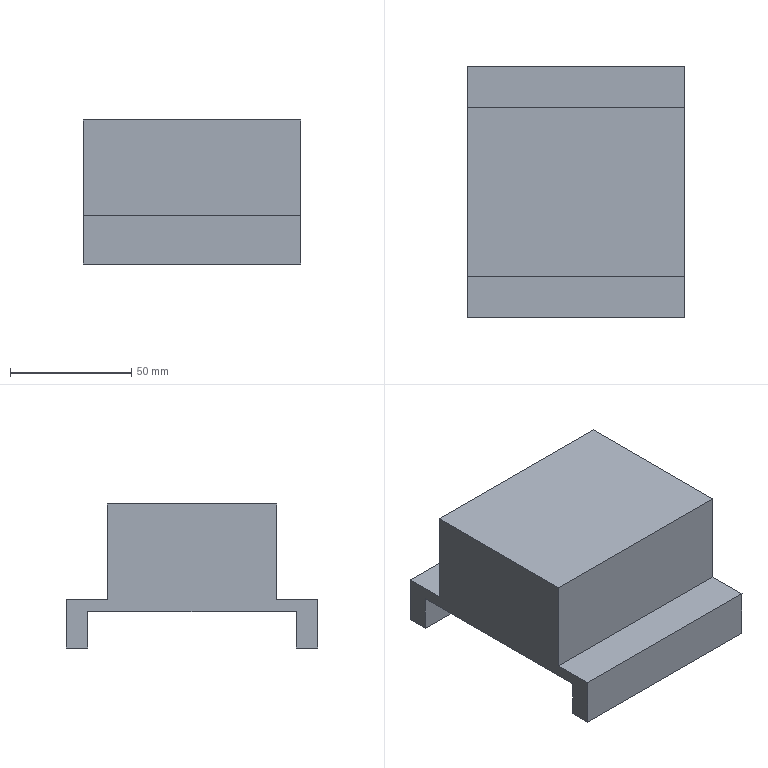Component | SolidWorks | X-AxisSlider-1 | 1 solid | 32 faces | box 90 x 104 x 59.5 mm | volume 318772 mm3 | plane 20 | cylinder 12 | commonest cylinder face diameters 5 x12
build123d program:
from build123d import *

# Parameters (mm, degrees)
BOSS_EXTRUDE1_DEPTH = 90
SKETCH3_R           = 2.5
CUT_EXTRUDE1_DEPTH  = 10


with BuildPart() as part:
    # Sketch2 → Boss-Extrude1 (new body)
    with BuildSketch(Plane.XY):
        Polygon((-35, 0), (35, 0), (35, 39.5), (52, 39.5), (52, 59.5), (43, 59.5), (43, 44.5), (-43, 44.5), (-43, 59.5), (-52, 59.5), (-52, 39.5), (-35, 39.5), align=None)
    extrude(amount=BOSS_EXTRUDE1_DEPTH)

    # Sketch3 → Cut-Extrude1 (cut)
    with BuildSketch(Plane(origin=(0, 59.5, 0), x_dir=(1, 0, 0), z_dir=(0, 1, 0))):
        with Locations(Location((-47.5, -8, 0), (0, 0, 180))):
            Circle(SKETCH3_R)
        with Locations(Location((-47.5, -45, 0), (0, 0, 180))):
            Circle(SKETCH3_R)
        with Locations(Location((-47.5, -82, 0), (0, 0, 180))):
            Circle(SKETCH3_R)
        with Locations(Location((47.5, -8, 0), (0, 0, 180))):
            Circle(SKETCH3_R)
        with Locations(Location((47.5, -45, 0), (0, 0, 180))):
            Circle(SKETCH3_R)
        with Locations(Location((47.5, -82, 0), (0, 0, 180))):
            Circle(SKETCH3_R)
    extrude(amount=-CUT_EXTRUDE1_DEPTH, mode=Mode.SUBTRACT)


solid = part.part

# Placed as in the assembly
solid = solid.moved(Location((-25.771, 0, 59), (-90, 90, 0)))
STEP:
#1=COLOUR_RGB('',0.7922,0.8196,0.9333);
#2=FILL_AREA_STYLE_COLOUR('',#1);
#3=FILL_AREA_STYLE('',(#2));
#4=SURFACE_STYLE_FILL_AREA(#3);
#5=SURFACE_SIDE_STYLE('',(#4));
#6=SURFACE_STYLE_USAGE(.BOTH.,#5);
#7=PRESENTATION_STYLE_ASSIGNMENT((#6));
#8=CARTESIAN_POINT('',(2.214,-1.969,0.374));
#9=VERTEX_POINT('',#8);
#10=CARTESIAN_POINT('',(2.214,-1.772,0.374));
#11=VERTEX_POINT('',#10);
#12=CARTESIAN_POINT('',(2.214,-1.87,0.374));
#13=DIRECTION('',(0.,0.,-1.));
#14=DIRECTION('',(0.,1.,0.));
#15=AXIS2_PLACEMENT_3D('',#12,#13,#14);
#16=CIRCLE('',#15,0.09843);
#17=EDGE_CURVE('',#9,#11,#16,.T.);
#18=ORIENTED_EDGE('',*,*,#17,.F.);
#19=CARTESIAN_POINT('',(2.214,-1.969,-0.01969));
#20=VERTEX_POINT('',#19);
#21=CARTESIAN_POINT('',(2.214,-1.969,0.374));
#22=DIRECTION('',(0.,0.,-1.));
#23=VECTOR('',#22,39.37);
#24=LINE('',#21,#23);
#25=EDGE_CURVE('',#9,#20,#24,.T.);
#26=ORIENTED_EDGE('',*,*,#25,.T.);
#27=CARTESIAN_POINT('',(2.214,-1.772,-0.01969));
#28=VERTEX_POINT('',#27);
#29=CARTESIAN_POINT('',(2.214,-1.87,-0.01969));
#30=DIRECTION('',(0.,0.,-1.));
#31=DIRECTION('',(0.,1.,0.));
#32=AXIS2_PLACEMENT_3D('',#29,#30,#31);
#33=CIRCLE('',#32,0.09843);
#34=EDGE_CURVE('',#20,#28,#33,.T.);
#35=ORIENTED_EDGE('',*,*,#34,.T.);
#36=CARTESIAN_POINT('',(2.214,-1.772,0.374));
#37=DIRECTION('',(0.,0.,-1.));
#38=VECTOR('',#37,39.37);
#39=LINE('',#36,#38);
#40=EDGE_CURVE('',#11,#28,#39,.T.);
#41=ORIENTED_EDGE('',*,*,#40,.F.);
#42=EDGE_LOOP('',(#18,#26,#35,#41));
#43=FACE_OUTER_BOUND('',#42,.T.);
#44=CARTESIAN_POINT('',(2.214,-1.87,0.374));
#45=DIRECTION('',(0.,0.,-1.));
#46=DIRECTION('',(0.,1.,0.));
#47=AXIS2_PLACEMENT_3D('',#44,#45,#46);
#48=CYLINDRICAL_SURFACE('',#47,0.09843);
#49=ADVANCED_FACE('',(#43),#48,.F.);
#50=CARTESIAN_POINT('',(0.7571,-1.969,0.374));
#51=VERTEX_POINT('',#50);
#52=CARTESIAN_POINT('',(0.7571,-1.772,0.374));
#53=VERTEX_POINT('',#52);
#54=CARTESIAN_POINT('',(0.7571,-1.87,0.374));
#55=DIRECTION('',(0.,0.,-1.));
#56=DIRECTION('',(0.,1.,0.));
#57=AXIS2_PLACEMENT_3D('',#54,#55,#56);
#58=CIRCLE('',#57,0.09843);
#59=EDGE_CURVE('',#51,#53,#58,.T.);
#60=ORIENTED_EDGE('',*,*,#59,.F.);
#61=CARTESIAN_POINT('',(0.7571,-1.969,-0.01969));
#62=VERTEX_POINT('',#61);
#63=CARTESIAN_POINT('',(0.7571,-1.969,0.374));
#64=DIRECTION('',(0.,0.,-1.));
#65=VECTOR('',#64,39.37);
#66=LINE('',#63,#65);
#67=EDGE_CURVE('',#51,#62,#66,.T.);
#68=ORIENTED_EDGE('',*,*,#67,.T.);
#69=CARTESIAN_POINT('',(0.7571,-1.772,-0.01969));
#70=VERTEX_POINT('',#69);
#71=CARTESIAN_POINT('',(0.7571,-1.87,-0.01969));
#72=DIRECTION('',(0.,0.,-1.));
#73=DIRECTION('',(0.,1.,0.));
#74=AXIS2_PLACEMENT_3D('',#71,#72,#73);
#75=CIRCLE('',#74,0.09843);
#76=EDGE_CURVE('',#62,#70,#75,.T.);
#77=ORIENTED_EDGE('',*,*,#76,.T.);
#78=CARTESIAN_POINT('',(0.7571,-1.772,0.374));
#79=DIRECTION('',(0.,0.,-1.));
#80=VECTOR('',#79,39.37);
#81=LINE('',#78,#80);
#82=EDGE_CURVE('',#53,#70,#81,.T.);
#83=ORIENTED_EDGE('',*,*,#82,.F.);
#84=EDGE_LOOP('',(#60,#68,#77,#83));
#85=FACE_OUTER_BOUND('',#84,.T.);
#86=CARTESIAN_POINT('',(0.7571,-1.87,0.374));
#87=DIRECTION('',(0.,0.,-1.));
#88=DIRECTION('',(0.,1.,0.));
#89=AXIS2_PLACEMENT_3D('',#86,#87,#88);
#90=CYLINDRICAL_SURFACE('',#89,0.09843);
#91=ADVANCED_FACE('',(#85),#90,.F.);
#92=CARTESIAN_POINT('',(-0.6996,-1.969,0.374));
#93=VERTEX_POINT('',#92);
#94=CARTESIAN_POINT('',(-0.6996,-1.772,0.374));
#95=VERTEX_POINT('',#94);
#96=CARTESIAN_POINT('',(-0.6996,-1.87,0.374));
#97=DIRECTION('',(0.,0.,-1.));
#98=DIRECTION('',(0.,1.,0.));
#99=AXIS2_PLACEMENT_3D('',#96,#97,#98);
#100=CIRCLE('',#99,0.09843);
#101=EDGE_CURVE('',#93,#95,#100,.T.);
#102=ORIENTED_EDGE('',*,*,#101,.F.);
#103=CARTESIAN_POINT('',(-0.6996,-1.969,-0.01969));
#104=VERTEX_POINT('',#103);
#105=CARTESIAN_POINT('',(-0.6996,-1.969,0.374));
#106=DIRECTION('',(0.,0.,-1.));
#107=VECTOR('',#106,39.37);
#108=LINE('',#105,#107);
#109=EDGE_CURVE('',#93,#104,#108,.T.);
#110=ORIENTED_EDGE('',*,*,#109,.T.);
#111=CARTESIAN_POINT('',(-0.6996,-1.772,-0.01969));
#112=VERTEX_POINT('',#111);
#113=CARTESIAN_POINT('',(-0.6996,-1.87,-0.01969));
#114=DIRECTION('',(0.,0.,-1.));
#115=DIRECTION('',(0.,1.,0.));
#116=AXIS2_PLACEMENT_3D('',#113,#114,#115);
#117=CIRCLE('',#116,0.09843);
#118=EDGE_CURVE('',#104,#112,#117,.T.);
#119=ORIENTED_EDGE('',*,*,#118,.T.);
#120=CARTESIAN_POINT('',(-0.6996,-1.772,0.374));
#121=DIRECTION('',(0.,0.,-1.));
#122=VECTOR('',#121,39.37);
#123=LINE('',#120,#122);
#124=EDGE_CURVE('',#95,#112,#123,.T.);
#125=ORIENTED_EDGE('',*,*,#124,.F.);
#126=EDGE_LOOP('',(#102,#110,#119,#125));
#127=FACE_OUTER_BOUND('',#126,.T.);
#128=CARTESIAN_POINT('',(-0.6996,-1.87,0.374));
#129=DIRECTION('',(0.,0.,-1.));
#130=DIRECTION('',(0.,1.,0.));
#131=AXIS2_PLACEMENT_3D('',#128,#129,#130);
#132=CYLINDRICAL_SURFACE('',#131,0.09843);
#133=ADVANCED_FACE('',(#127),#132,.F.);
#134=CARTESIAN_POINT('',(2.214,1.772,0.374));
#135=VERTEX_POINT('',#134);
#136=CARTESIAN_POINT('',(2.214,1.969,0.374));
#137=VERTEX_POINT('',#136);
#138=CARTESIAN_POINT('',(2.214,1.87,0.374));
#139=DIRECTION('',(0.,0.,-1.));
#140=DIRECTION('',(0.,1.,0.));
#141=AXIS2_PLACEMENT_3D('',#138,#139,#140);
#142=CIRCLE('',#141,0.09843);
#143=EDGE_CURVE('',#135,#137,#142,.T.);
#144=ORIENTED_EDGE('',*,*,#143,.F.);
#145=CARTESIAN_POINT('',(2.214,1.772,-0.01969));
#146=VERTEX_POINT('',#145);
#147=CARTESIAN_POINT('',(2.214,1.772,0.374));
#148=DIRECTION('',(0.,0.,-1.));
#149=VECTOR('',#148,39.37);
#150=LINE('',#147,#149);
#151=EDGE_CURVE('',#135,#146,#150,.T.);
#152=ORIENTED_EDGE('',*,*,#151,.T.);
#153=CARTESIAN_POINT('',(2.214,1.969,-0.01969));
#154=VERTEX_POINT('',#153);
#155=CARTESIAN_POINT('',(2.214,1.87,-0.01969));
#156=DIRECTION('',(0.,0.,-1.));
#157=DIRECTION('',(0.,1.,0.));
#158=AXIS2_PLACEMENT_3D('',#155,#156,#157);
#159=CIRCLE('',#158,0.09843);
#160=EDGE_CURVE('',#146,#154,#159,.T.);
#161=ORIENTED_EDGE('',*,*,#160,.T.);
#162=CARTESIAN_POINT('',(2.214,1.969,0.374));
#163=DIRECTION('',(0.,0.,-1.));
#164=VECTOR('',#163,39.37);
#165=LINE('',#162,#164);
#166=EDGE_CURVE('',#137,#154,#165,.T.);
#167=ORIENTED_EDGE('',*,*,#166,.F.);
#168=EDGE_LOOP('',(#144,#152,#161,#167));
#169=FACE_OUTER_BOUND('',#168,.T.);
#170=CARTESIAN_POINT('',(2.214,1.87,0.374));
#171=DIRECTION('',(0.,0.,-1.));
#172=DIRECTION('',(0.,1.,0.));
#173=AXIS2_PLACEMENT_3D('',#170,#171,#172);
#174=CYLINDRICAL_SURFACE('',#173,0.09843);
#175=ADVANCED_FACE('',(#169),#174,.F.);
#176=CARTESIAN_POINT('',(0.7571,1.772,0.374));
#177=VERTEX_POINT('',#176);
#178=CARTESIAN_POINT('',(0.7571,1.969,0.374));
#179=VERTEX_POINT('',#178);
#180=CARTESIAN_POINT('',(0.7571,1.87,0.374));
#181=DIRECTION('',(0.,0.,-1.));
#182=DIRECTION('',(0.,1.,0.));
#183=AXIS2_PLACEMENT_3D('',#180,#181,#182);
#184=CIRCLE('',#183,0.09843);
#185=EDGE_CURVE('',#177,#179,#184,.T.);
#186=ORIENTED_EDGE('',*,*,#185,.F.);
#187=CARTESIAN_POINT('',(0.7571,1.772,-0.01969));
#188=VERTEX_POINT('',#187);
#189=CARTESIAN_POINT('',(0.7571,1.772,0.374));
#190=DIRECTION('',(0.,0.,-1.));
#191=VECTOR('',#190,39.37);
#192=LINE('',#189,#191);
#193=EDGE_CURVE('',#177,#188,#192,.T.);
#194=ORIENTED_EDGE('',*,*,#193,.T.);
#195=CARTESIAN_POINT('',(0.7571,1.969,-0.01969));
#196=VERTEX_POINT('',#195);
#197=CARTESIAN_POINT('',(0.7571,1.87,-0.01969));
#198=DIRECTION('',(0.,0.,-1.));
#199=DIRECTION('',(0.,1.,0.));
#200=AXIS2_PLACEMENT_3D('',#197,#198,#199);
#201=CIRCLE('',#200,0.09843);
#202=EDGE_CURVE('',#188,#196,#201,.T.);
#203=ORIENTED_EDGE('',*,*,#202,.T.);
#204=CARTESIAN_POINT('',(0.7571,1.969,0.374));
#205=DIRECTION('',(0.,0.,-1.));
#206=VECTOR('',#205,39.37);
#207=LINE('',#204,#206);
#208=EDGE_CURVE('',#179,#196,#207,.T.);
#209=ORIENTED_EDGE('',*,*,#208,.F.);
#210=EDGE_LOOP('',(#186,#194,#203,#209));
#211=FACE_OUTER_BOUND('',#210,.T.);
#212=CARTESIAN_POINT('',(0.7571,1.87,0.374));
#213=DIRECTION('',(0.,0.,-1.));
#214=DIRECTION('',(0.,1.,0.));
#215=AXIS2_PLACEMENT_3D('',#212,#213,#214);
#216=CYLINDRICAL_SURFACE('',#215,0.09843);
#217=ADVANCED_FACE('',(#211),#216,.F.);
#218=CARTESIAN_POINT('',(-0.6996,1.772,0.374));
#219=VERTEX_POINT('',#218);
#220=CARTESIAN_POINT('',(-0.6996,1.969,0.374));
#221=VERTEX_POINT('',#220);
#222=CARTESIAN_POINT('',(-0.6996,1.87,0.374));
#223=DIRECTION('',(0.,0.,-1.));
#224=DIRECTION('',(0.,1.,0.));
#225=AXIS2_PLACEMENT_3D('',#222,#223,#224);
#226=CIRCLE('',#225,0.09843);
#227=EDGE_CURVE('',#219,#221,#226,.T.);
#228=ORIENTED_EDGE('',*,*,#227,.F.);
#229=CARTESIAN_POINT('',(-0.6996,1.772,-0.01969));
#230=VERTEX_POINT('',#229);
#231=CARTESIAN_POINT('',(-0.6996,1.772,0.374));
#232=DIRECTION('',(0.,0.,-1.));
#233=VECTOR('',#232,39.37);
#234=LINE('',#231,#233);
#235=EDGE_CURVE('',#219,#230,#234,.T.);
#236=ORIENTED_EDGE('',*,*,#235,.T.);
#237=CARTESIAN_POINT('',(-0.6996,1.969,-0.01969));
#238=VERTEX_POINT('',#237);
#239=CARTESIAN_POINT('',(-0.6996,1.87,-0.01969));
#240=DIRECTION('',(0.,0.,-1.));
#241=DIRECTION('',(0.,1.,0.));
#242=AXIS2_PLACEMENT_3D('',#239,#240,#241);
#243=CIRCLE('',#242,0.09843);
#244=EDGE_CURVE('',#230,#238,#243,.T.);
#245=ORIENTED_EDGE('',*,*,#244,.T.);
#246=CARTESIAN_POINT('',(-0.6996,1.969,0.374));
#247=DIRECTION('',(0.,0.,-1.));
#248=VECTOR('',#247,39.37);
#249=LINE('',#246,#248);
#250=EDGE_CURVE('',#221,#238,#249,.T.);
#251=ORIENTED_EDGE('',*,*,#250,.F.);
#252=EDGE_LOOP('',(#228,#236,#245,#251));
#253=FACE_OUTER_BOUND('',#252,.T.);
#254=CARTESIAN_POINT('',(-0.6996,1.87,0.374));
#255=DIRECTION('',(0.,0.,-1.));
#256=DIRECTION('',(0.,1.,0.));
#257=AXIS2_PLACEMENT_3D('',#254,#255,#256);
#258=CYLINDRICAL_SURFACE('',#257,0.09843);
#259=ADVANCED_FACE('',(#253),#258,.F.);
#260=CARTESIAN_POINT('',(-1.015,1.378,0.7677));
#261=VERTEX_POINT('',#260);
#262=CARTESIAN_POINT('',(-1.015,1.378,2.323));
#263=VERTEX_POINT('',#262);
#264=CARTESIAN_POINT('',(-1.015,1.378,2.323));
#265=DIRECTION('',(-0.,-0.,1.));
#266=VECTOR('',#265,39.37);
#267=LINE('',#264,#266);
#268=EDGE_CURVE('',#261,#263,#267,.T.);
#269=ORIENTED_EDGE('',*,*,#268,.T.);
#270=CARTESIAN_POINT('',(2.529,1.378,2.323));
#271=VERTEX_POINT('',#270);
#272=CARTESIAN_POINT('',(2.529,1.378,2.323));
#273=DIRECTION('',(-1.,-0.,-0.));
#274=VECTOR('',#273,39.37);
#275=LINE('',#272,#274);
#276=EDGE_CURVE('',#271,#263,#275,.T.);
#277=ORIENTED_EDGE('',*,*,#276,.F.);
#278=CARTESIAN_POINT('',(2.529,1.378,0.7677));
#279=VERTEX_POINT('',#278);
#280=CARTESIAN_POINT('',(2.529,1.378,2.323));
#281=DIRECTION('',(-0.,-0.,1.));
#282=VECTOR('',#281,39.37);
#283=LINE('',#280,#282);
#284=EDGE_CURVE('',#279,#271,#283,.T.);
#285=ORIENTED_EDGE('',*,*,#284,.F.);
#286=CARTESIAN_POINT('',(2.529,1.378,0.7677));
#287=DIRECTION('',(-1.,-0.,-0.));
#288=VECTOR('',#287,39.37);
#289=LINE('',#286,#288);
#290=EDGE_CURVE('',#279,#261,#289,.T.);
#291=ORIENTED_EDGE('',*,*,#290,.T.);
#292=EDGE_LOOP('',(#269,#277,#285,#291));
#293=FACE_OUTER_BOUND('',#292,.T.);
#294=CARTESIAN_POINT('',(2.529,1.378,2.323));
#295=DIRECTION('',(0.,-1.,-0.));
#296=DIRECTION('',(-1.,-0.,-0.));
#297=AXIS2_PLACEMENT_3D('',#294,#295,#296);
#298=PLANE('',#297);
#299=ADVANCED_FACE('',(#293),#298,.F.);
#300=CARTESIAN_POINT('',(-1.015,-1.378,2.323));
#301=VERTEX_POINT('',#300);
#302=CARTESIAN_POINT('',(-1.015,1.378,2.323));
#303=DIRECTION('',(0.,-1.,-0.));
#304=VECTOR('',#303,39.37);
#305=LINE('',#302,#304);
#306=EDGE_CURVE('',#263,#301,#305,.T.);
#307=ORIENTED_EDGE('',*,*,#306,.T.);
#308=CARTESIAN_POINT('',(2.529,-1.378,2.323));
#309=VERTEX_POINT('',#308);
#310=CARTESIAN_POINT('',(2.529,-1.378,2.323));
#311=DIRECTION('',(-1.,-0.,-0.));
#312=VECTOR('',#311,39.37);
#313=LINE('',#310,#312);
#314=EDGE_CURVE('',#309,#301,#313,.T.);
#315=ORIENTED_EDGE('',*,*,#314,.F.);
#316=CARTESIAN_POINT('',(2.529,1.378,2.323));
#317=DIRECTION('',(0.,-1.,-0.));
#318=VECTOR('',#317,39.37);
#319=LINE('',#316,#318);
#320=EDGE_CURVE('',#271,#309,#319,.T.);
#321=ORIENTED_EDGE('',*,*,#320,.F.);
#322=ORIENTED_EDGE('',*,*,#276,.T.);
#323=EDGE_LOOP('',(#307,#315,#321,#322));
#324=FACE_OUTER_BOUND('',#323,.T.);
#325=CARTESIAN_POINT('',(2.529,1.378,2.323));
#326=DIRECTION('',(0.,0.,-1.));
#327=DIRECTION('',(1.,0.,0.));
#328=AXIS2_PLACEMENT_3D('',#325,#326,#327);
#329=PLANE('',#328);
#330=ADVANCED_FACE('',(#324),#329,.F.);
#331=CARTESIAN_POINT('',(-1.015,-1.378,0.7677));
#332=VERTEX_POINT('',#331);
#333=CARTESIAN_POINT('',(-1.015,-1.378,2.323));
#334=DIRECTION('',(0.,0.,-1.));
#335=VECTOR('',#334,39.37);
#336=LINE('',#333,#335);
#337=EDGE_CURVE('',#301,#332,#336,.T.);
#338=ORIENTED_EDGE('',*,*,#337,.T.);
#339=CARTESIAN_POINT('',(2.529,-1.378,0.7677));
#340=VERTEX_POINT('',#339);
#341=CARTESIAN_POINT('',(2.529,-1.378,0.7677));
#342=DIRECTION('',(-1.,-0.,-0.));
#343=VECTOR('',#342,39.37);
#344=LINE('',#341,#343);
#345=EDGE_CURVE('',#340,#332,#344,.T.);
#346=ORIENTED_EDGE('',*,*,#345,.F.);
#347=CARTESIAN_POINT('',(2.529,-1.378,2.323));
#348=DIRECTION('',(0.,0.,-1.));
#349=VECTOR('',#348,39.37);
#350=LINE('',#347,#349);
#351=EDGE_CURVE('',#309,#340,#350,.T.);
#352=ORIENTED_EDGE('',*,*,#351,.F.);
#353=ORIENTED_EDGE('',*,*,#314,.T.);
#354=EDGE_LOOP('',(#338,#346,#352,#353));
#355=FACE_OUTER_BOUND('',#354,.T.);
#356=CARTESIAN_POINT('',(2.529,-1.378,2.323));
#357=DIRECTION('',(-0.,1.,0.));
#358=DIRECTION('',(1.,0.,0.));
#359=AXIS2_PLACEMENT_3D('',#356,#357,#358);
#360=PLANE('',#359);
#361=ADVANCED_FACE('',(#355),#360,.F.);
#362=CARTESIAN_POINT('',(-1.015,-2.047,0.7677));
#363=VERTEX_POINT('',#362);
#364=CARTESIAN_POINT('',(-1.015,-1.378,0.7677));
#365=DIRECTION('',(0.,-1.,-0.));
#366=VECTOR('',#365,39.37);
#367=LINE('',#364,#366);
#368=EDGE_CURVE('',#332,#363,#367,.T.);
#369=ORIENTED_EDGE('',*,*,#368,.T.);
#370=CARTESIAN_POINT('',(2.529,-2.047,0.7677));
#371=VERTEX_POINT('',#370);
#372=CARTESIAN_POINT('',(2.529,-2.047,0.7677));
#373=DIRECTION('',(-1.,-0.,-0.));
#374=VECTOR('',#373,39.37);
#375=LINE('',#372,#374);
#376=EDGE_CURVE('',#371,#363,#375,.T.);
#377=ORIENTED_EDGE('',*,*,#376,.F.);
#378=CARTESIAN_POINT('',(2.529,-1.378,0.7677));
#379=DIRECTION('',(0.,-1.,-0.));
#380=VECTOR('',#379,39.37);
#381=LINE('',#378,#380);
#382=EDGE_CURVE('',#340,#371,#381,.T.);
#383=ORIENTED_EDGE('',*,*,#382,.F.);
#384=ORIENTED_EDGE('',*,*,#345,.T.);
#385=EDGE_LOOP('',(#369,#377,#383,#384));
#386=FACE_OUTER_BOUND('',#385,.T.);
#387=CARTESIAN_POINT('',(2.529,-1.378,0.7677));
#388=DIRECTION('',(0.,0.,-1.));
#389=DIRECTION('',(1.,0.,0.));
#390=AXIS2_PLACEMENT_3D('',#387,#388,#389);
#391=PLANE('',#390);
#392=ADVANCED_FACE('',(#386),#391,.F.);
#393=CARTESIAN_POINT('',(-1.015,-2.047,-0.01969));
#394=VERTEX_POINT('',#393);
#395=CARTESIAN_POINT('',(-1.015,-2.047,0.7677));
#396=DIRECTION('',(0.,0.,-1.));
#397=VECTOR('',#396,39.37);
#398=LINE('',#395,#397);
#399=EDGE_CURVE('',#363,#394,#398,.T.);
#400=ORIENTED_EDGE('',*,*,#399,.T.);
#401=CARTESIAN_POINT('',(2.529,-2.047,-0.01969));
#402=VERTEX_POINT('',#401);
#403=CARTESIAN_POINT('',(2.529,-2.047,-0.01969));
#404=DIRECTION('',(-1.,-0.,-0.));
#405=VECTOR('',#404,39.37);
#406=LINE('',#403,#405);
#407=EDGE_CURVE('',#402,#394,#406,.T.);
#408=ORIENTED_EDGE('',*,*,#407,.F.);
#409=CARTESIAN_POINT('',(2.529,-2.047,0.7677));
#410=DIRECTION('',(0.,0.,-1.));
#411=VECTOR('',#410,39.37);
#412=LINE('',#409,#411);
#413=EDGE_CURVE('',#371,#402,#412,.T.);
#414=ORIENTED_EDGE('',*,*,#413,.F.);
#415=ORIENTED_EDGE('',*,*,#376,.T.);
#416=EDGE_LOOP('',(#400,#408,#414,#415));
#417=FACE_OUTER_BOUND('',#416,.T.);
#418=CARTESIAN_POINT('',(2.529,-2.047,0.7677));
#419=DIRECTION('',(-0.,1.,0.));
#420=DIRECTION('',(1.,0.,0.));
#421=AXIS2_PLACEMENT_3D('',#418,#419,#420);
#422=PLANE('',#421);
#423=ADVANCED_FACE('',(#417),#422,.F.);
#424=CARTESIAN_POINT('',(2.214,-1.87,-0.01969));
#425=DIRECTION('',(0.,0.,-1.));
#426=DIRECTION('',(0.,1.,0.));
#427=AXIS2_PLACEMENT_3D('',#424,#425,#426);
#428=CIRCLE('',#427,0.09843);
#429=EDGE_CURVE('',#28,#20,#428,.T.);
#430=ORIENTED_EDGE('',*,*,#429,.F.);
#431=ORIENTED_EDGE('',*,*,#34,.F.);
#432=EDGE_LOOP('',(#430,#431));
#433=FACE_BOUND('',#432,.T.);
#434=CARTESIAN_POINT('',(0.7571,-1.87,-0.01969));
#435=DIRECTION('',(0.,0.,-1.));
#436=DIRECTION('',(0.,1.,0.));
#437=AXIS2_PLACEMENT_3D('',#434,#435,#436);
#438=CIRCLE('',#437,0.09843);
#439=EDGE_CURVE('',#70,#62,#438,.T.);
#440=ORIENTED_EDGE('',*,*,#439,.F.);
#441=ORIENTED_EDGE('',*,*,#76,.F.);
#442=EDGE_LOOP('',(#440,#441));
#443=FACE_BOUND('',#442,.T.);
#444=CARTESIAN_POINT('',(-0.6996,-1.87,-0.01969));
#445=DIRECTION('',(0.,0.,-1.));
#446=DIRECTION('',(0.,1.,0.));
#447=AXIS2_PLACEMENT_3D('',#444,#445,#446);
#448=CIRCLE('',#447,0.09843);
#449=EDGE_CURVE('',#112,#104,#448,.T.);
#450=ORIENTED_EDGE('',*,*,#449,.F.);
#451=ORIENTED_EDGE('',*,*,#118,.F.);
#452=EDGE_LOOP('',(#450,#451));
#453=FACE_BOUND('',#452,.T.);
#454=CARTESIAN_POINT('',(-1.015,-1.693,-0.01969));
#455=VERTEX_POINT('',#454);
#456=CARTESIAN_POINT('',(-1.015,-2.047,-0.01969));
#457=DIRECTION('',(-0.,1.,0.));
#458=VECTOR('',#457,39.37);
#459=LINE('',#456,#458);
#460=EDGE_CURVE('',#394,#455,#459,.T.);
#461=ORIENTED_EDGE('',*,*,#460,.T.);
#462=CARTESIAN_POINT('',(2.529,-1.693,-0.01969));
#463=VERTEX_POINT('',#462);
#464=CARTESIAN_POINT('',(2.529,-1.693,-0.01969));
#465=DIRECTION('',(-1.,-0.,-0.));
#466=VECTOR('',#465,39.37);
#467=LINE('',#464,#466);
#468=EDGE_CURVE('',#463,#455,#467,.T.);
#469=ORIENTED_EDGE('',*,*,#468,.F.);
#470=CARTESIAN_POINT('',(2.529,-2.047,-0.01969));
#471=DIRECTION('',(-0.,1.,0.));
#472=VECTOR('',#471,39.37);
#473=LINE('',#470,#472);
#474=EDGE_CURVE('',#402,#463,#473,.T.);
#475=ORIENTED_EDGE('',*,*,#474,.F.);
#476=ORIENTED_EDGE('',*,*,#407,.T.);
#477=EDGE_LOOP('',(#461,#469,#475,#476));
#478=FACE_OUTER_BOUND('',#477,.T.);
#479=CARTESIAN_POINT('',(2.529,-2.047,-0.01969));
#480=DIRECTION('',(-0.,-0.,1.));
#481=DIRECTION('',(0.,-1.,-0.));
#482=AXIS2_PLACEMENT_3D('',#479,#480,#481);
#483=PLANE('',#482);
#484=ADVANCED_FACE('',(#433,#443,#453,#478),#483,.F.);
#485=CARTESIAN_POINT('',(-1.015,-1.693,0.5709));
#486=VERTEX_POINT('',#485);
#487=CARTESIAN_POINT('',(-1.015,-1.693,-0.01969));
#488=DIRECTION('',(-0.,-0.,1.));
#489=VECTOR('',#488,39.37);
#490=LINE('',#487,#489);
#491=EDGE_CURVE('',#455,#486,#490,.T.);
#492=ORIENTED_EDGE('',*,*,#491,.T.);
#493=CARTESIAN_POINT('',(2.529,-1.693,0.5709));
#494=VERTEX_POINT('',#493);
#495=CARTESIAN_POINT('',(2.529,-1.693,0.5709));
#496=DIRECTION('',(-1.,-0.,-0.));
#497=VECTOR('',#496,39.37);
#498=LINE('',#495,#497);
#499=EDGE_CURVE('',#494,#486,#498,.T.);
#500=ORIENTED_EDGE('',*,*,#499,.F.);
#501=CARTESIAN_POINT('',(2.529,-1.693,-0.01969));
#502=DIRECTION('',(-0.,-0.,1.));
#503=VECTOR('',#502,39.37);
#504=LINE('',#501,#503);
#505=EDGE_CURVE('',#463,#494,#504,.T.);
#506=ORIENTED_EDGE('',*,*,#505,.F.);
#507=ORIENTED_EDGE('',*,*,#468,.T.);
#508=EDGE_LOOP('',(#492,#500,#506,#507));
#509=FACE_OUTER_BOUND('',#508,.T.);
#510=CARTESIAN_POINT('',(2.529,-1.693,-0.01969));
#511=DIRECTION('',(0.,-1.,-0.));
#512=DIRECTION('',(-1.,-0.,-0.));
#513=AXIS2_PLACEMENT_3D('',#510,#511,#512);
#514=PLANE('',#513);
#515=ADVANCED_FACE('',(#509),#514,.F.);
#516=CARTESIAN_POINT('',(-1.015,1.693,0.5709));
#517=VERTEX_POINT('',#516);
#518=CARTESIAN_POINT('',(-1.015,-1.693,0.5709));
#519=DIRECTION('',(-0.,1.,0.));
#520=VECTOR('',#519,39.37);
#521=LINE('',#518,#520);
#522=EDGE_CURVE('',#486,#517,#521,.T.);
#523=ORIENTED_EDGE('',*,*,#522,.T.);
#524=CARTESIAN_POINT('',(2.529,1.693,0.5709));
#525=VERTEX_POINT('',#524);
#526=CARTESIAN_POINT('',(2.529,1.693,0.5709));
#527=DIRECTION('',(-1.,-0.,-0.));
#528=VECTOR('',#527,39.37);
#529=LINE('',#526,#528);
#530=EDGE_CURVE('',#525,#517,#529,.T.);
#531=ORIENTED_EDGE('',*,*,#530,.F.);
#532=CARTESIAN_POINT('',(2.529,-1.693,0.5709));
#533=DIRECTION('',(-0.,1.,0.));
#534=VECTOR('',#533,39.37);
#535=LINE('',#532,#534);
#536=EDGE_CURVE('',#494,#525,#535,.T.);
#537=ORIENTED_EDGE('',*,*,#536,.F.);
#538=ORIENTED_EDGE('',*,*,#499,.T.);
#539=EDGE_LOOP('',(#523,#531,#537,#538));
#540=FACE_OUTER_BOUND('',#539,.T.);
#541=CARTESIAN_POINT('',(2.529,-1.693,0.5709));
#542=DIRECTION('',(-0.,-0.,1.));
#543=DIRECTION('',(0.,-1.,-0.));
#544=AXIS2_PLACEMENT_3D('',#541,#542,#543);
#545=PLANE('',#544);
#546=ADVANCED_FACE('',(#540),#545,.F.);
#547=CARTESIAN_POINT('',(-1.015,1.693,-0.01969));
#548=VERTEX_POINT('',#547);
#549=CARTESIAN_POINT('',(-1.015,1.693,0.5709));
#550=DIRECTION('',(0.,0.,-1.));
#551=VECTOR('',#550,39.37);
#552=LINE('',#549,#551);
#553=EDGE_CURVE('',#517,#548,#552,.T.);
#554=ORIENTED_EDGE('',*,*,#553,.T.);
#555=CARTESIAN_POINT('',(2.529,1.693,-0.01969));
#556=VERTEX_POINT('',#555);
#557=CARTESIAN_POINT('',(2.529,1.693,-0.01969));
#558=DIRECTION('',(-1.,-0.,-0.));
#559=VECTOR('',#558,39.37);
#560=LINE('',#557,#559);
#561=EDGE_CURVE('',#556,#548,#560,.T.);
#562=ORIENTED_EDGE('',*,*,#561,.F.);
#563=CARTESIAN_POINT('',(2.529,1.693,0.5709));
#564=DIRECTION('',(0.,0.,-1.));
#565=VECTOR('',#564,39.37);
#566=LINE('',#563,#565);
#567=EDGE_CURVE('',#525,#556,#566,.T.);
#568=ORIENTED_EDGE('',*,*,#567,.F.);
#569=ORIENTED_EDGE('',*,*,#530,.T.);
#570=EDGE_LOOP('',(#554,#562,#568,#569));
#571=FACE_OUTER_BOUND('',#570,.T.);
#572=CARTESIAN_POINT('',(2.529,1.693,0.5709));
#573=DIRECTION('',(-0.,1.,0.));
#574=DIRECTION('',(-0.,-0.,1.));
#575=AXIS2_PLACEMENT_3D('',#572,#573,#574);
#576=PLANE('',#575);
#577=ADVANCED_FACE('',(#571),#576,.F.);
#578=CARTESIAN_POINT('',(2.214,1.87,-0.01969));
#579=DIRECTION('',(0.,0.,-1.));
#580=DIRECTION('',(0.,1.,0.));
#581=AXIS2_PLACEMENT_3D('',#578,#579,#580);
#582=CIRCLE('',#581,0.09843);
#583=EDGE_CURVE('',#154,#146,#582,.T.);
#584=ORIENTED_EDGE('',*,*,#583,.F.);
#585=ORIENTED_EDGE('',*,*,#160,.F.);
#586=EDGE_LOOP('',(#584,#585));
#587=FACE_BOUND('',#586,.T.);
#588=CARTESIAN_POINT('',(0.7571,1.87,-0.01969));
#589=DIRECTION('',(0.,0.,-1.));
#590=DIRECTION('',(0.,1.,0.));
#591=AXIS2_PLACEMENT_3D('',#588,#589,#590);
#592=CIRCLE('',#591,0.09843);
#593=EDGE_CURVE('',#196,#188,#592,.T.);
#594=ORIENTED_EDGE('',*,*,#593,.F.);
#595=ORIENTED_EDGE('',*,*,#202,.F.);
#596=EDGE_LOOP('',(#594,#595));
#597=FACE_BOUND('',#596,.T.);
#598=CARTESIAN_POINT('',(-0.6996,1.87,-0.01969));
#599=DIRECTION('',(0.,0.,-1.));
#600=DIRECTION('',(0.,1.,0.));
#601=AXIS2_PLACEMENT_3D('',#598,#599,#600);
#602=CIRCLE('',#601,0.09843);
#603=EDGE_CURVE('',#238,#230,#602,.T.);
#604=ORIENTED_EDGE('',*,*,#603,.F.);
#605=ORIENTED_EDGE('',*,*,#244,.F.);
#606=EDGE_LOOP('',(#604,#605));
#607=FACE_BOUND('',#606,.T.);
#608=CARTESIAN_POINT('',(-1.015,2.047,-0.01969));
#609=VERTEX_POINT('',#608);
#610=CARTESIAN_POINT('',(-1.015,1.693,-0.01969));
#611=DIRECTION('',(-0.,1.,0.));
#612=VECTOR('',#611,39.37);
#613=LINE('',#610,#612);
#614=EDGE_CURVE('',#548,#609,#613,.T.);
#615=ORIENTED_EDGE('',*,*,#614,.T.);
#616=CARTESIAN_POINT('',(2.529,2.047,-0.01969));
#617=VERTEX_POINT('',#616);
#618=CARTESIAN_POINT('',(2.529,2.047,-0.01969));
#619=DIRECTION('',(-1.,-0.,-0.));
#620=VECTOR('',#619,39.37);
#621=LINE('',#618,#620);
#622=EDGE_CURVE('',#617,#609,#621,.T.);
#623=ORIENTED_EDGE('',*,*,#622,.F.);
#624=CARTESIAN_POINT('',(2.529,1.693,-0.01969));
#625=DIRECTION('',(-0.,1.,0.));
#626=VECTOR('',#625,39.37);
#627=LINE('',#624,#626);
#628=EDGE_CURVE('',#556,#617,#627,.T.);
#629=ORIENTED_EDGE('',*,*,#628,.F.);
#630=ORIENTED_EDGE('',*,*,#561,.T.);
#631=EDGE_LOOP('',(#615,#623,#629,#630));
#632=FACE_OUTER_BOUND('',#631,.T.);
#633=CARTESIAN_POINT('',(2.529,1.693,-0.01969));
#634=DIRECTION('',(-0.,-0.,1.));
#635=DIRECTION('',(-1.,-0.,-0.));
#636=AXIS2_PLACEMENT_3D('',#633,#634,#635);
#637=PLANE('',#636);
#638=ADVANCED_FACE('',(#587,#597,#607,#632),#637,.F.);
#639=CARTESIAN_POINT('',(-1.015,2.047,0.7677));
#640=VERTEX_POINT('',#639);
#641=CARTESIAN_POINT('',(-1.015,2.047,-0.01969));
#642=DIRECTION('',(-0.,-0.,1.));
#643=VECTOR('',#642,39.37);
#644=LINE('',#641,#643);
#645=EDGE_CURVE('',#609,#640,#644,.T.);
#646=ORIENTED_EDGE('',*,*,#645,.T.);
#647=CARTESIAN_POINT('',(2.529,2.047,0.7677));
#648=VERTEX_POINT('',#647);
#649=CARTESIAN_POINT('',(2.529,2.047,0.7677));
#650=DIRECTION('',(-1.,-0.,-0.));
#651=VECTOR('',#650,39.37);
#652=LINE('',#649,#651);
#653=EDGE_CURVE('',#648,#640,#652,.T.);
#654=ORIENTED_EDGE('',*,*,#653,.F.);
#655=CARTESIAN_POINT('',(2.529,2.047,-0.01969));
#656=DIRECTION('',(-0.,-0.,1.));
#657=VECTOR('',#656,39.37);
#658=LINE('',#655,#657);
#659=EDGE_CURVE('',#617,#648,#658,.T.);
#660=ORIENTED_EDGE('',*,*,#659,.F.);
#661=ORIENTED_EDGE('',*,*,#622,.T.);
#662=EDGE_LOOP('',(#646,#654,#660,#661));
#663=FACE_OUTER_BOUND('',#662,.T.);
#664=CARTESIAN_POINT('',(2.529,2.047,-0.01969));
#665=DIRECTION('',(0.,-1.,-0.));
#666=DIRECTION('',(-1.,-0.,-0.));
#667=AXIS2_PLACEMENT_3D('',#664,#665,#666);
#668=PLANE('',#667);
#669=ADVANCED_FACE('',(#663),#668,.F.);
#670=CARTESIAN_POINT('',(-1.015,2.047,0.7677));
#671=DIRECTION('',(0.,-1.,-0.));
#672=VECTOR('',#671,39.37);
#673=LINE('',#670,#672);
#674=EDGE_CURVE('',#640,#261,#673,.T.);
#675=ORIENTED_EDGE('',*,*,#674,.T.);
#676=ORIENTED_EDGE('',*,*,#290,.F.);
#677=CARTESIAN_POINT('',(2.529,2.047,0.7677));
#678=DIRECTION('',(0.,-1.,-0.));
#679=VECTOR('',#678,39.37);
#680=LINE('',#677,#679);
#681=EDGE_CURVE('',#648,#279,#680,.T.);
#682=ORIENTED_EDGE('',*,*,#681,.F.);
#683=ORIENTED_EDGE('',*,*,#653,.T.);
#684=EDGE_LOOP('',(#675,#676,#682,#683));
#685=FACE_OUTER_BOUND('',#684,.T.);
#686=CARTESIAN_POINT('',(2.529,2.047,0.7677));
#687=DIRECTION('',(0.,0.,-1.));
#688=DIRECTION('',(1.,0.,0.));
#689=AXIS2_PLACEMENT_3D('',#686,#687,#688);
#690=PLANE('',#689);
#691=ADVANCED_FACE('',(#685),#690,.F.);
#692=ORIENTED_EDGE('',*,*,#284,.T.);
#693=ORIENTED_EDGE('',*,*,#320,.T.);
#694=ORIENTED_EDGE('',*,*,#351,.T.);
#695=ORIENTED_EDGE('',*,*,#382,.T.);
#696=ORIENTED_EDGE('',*,*,#413,.T.);
#697=ORIENTED_EDGE('',*,*,#474,.T.);
#698=ORIENTED_EDGE('',*,*,#505,.T.);
#699=ORIENTED_EDGE('',*,*,#536,.T.);
#700=ORIENTED_EDGE('',*,*,#567,.T.);
#701=ORIENTED_EDGE('',*,*,#628,.T.);
#702=ORIENTED_EDGE('',*,*,#659,.T.);
#703=ORIENTED_EDGE('',*,*,#681,.T.);
#704=EDGE_LOOP('',(#692,#693,#694,#695,#696,#697,#698,#699,#700,#701,#702,#703));
#705=FACE_OUTER_BOUND('',#704,.T.);
#706=CARTESIAN_POINT('',(2.529,-0.,2.323));
#707=DIRECTION('',(-1.,-0.,-0.));
#708=DIRECTION('',(-0.,1.,0.));
#709=AXIS2_PLACEMENT_3D('',#706,#707,#708);
#710=PLANE('',#709);
#711=ADVANCED_FACE('',(#705),#710,.F.);
#712=ORIENTED_EDGE('',*,*,#268,.F.);
#713=ORIENTED_EDGE('',*,*,#674,.F.);
#714=ORIENTED_EDGE('',*,*,#645,.F.);
#715=ORIENTED_EDGE('',*,*,#614,.F.);
#716=ORIENTED_EDGE('',*,*,#553,.F.);
#717=ORIENTED_EDGE('',*,*,#522,.F.);
#718=ORIENTED_EDGE('',*,*,#491,.F.);
#719=ORIENTED_EDGE('',*,*,#460,.F.);
#720=ORIENTED_EDGE('',*,*,#399,.F.);
#721=ORIENTED_EDGE('',*,*,#368,.F.);
#722=ORIENTED_EDGE('',*,*,#337,.F.);
#723=ORIENTED_EDGE('',*,*,#306,.F.);
#724=EDGE_LOOP('',(#712,#713,#714,#715,#716,#717,#718,#719,#720,#721,#722,#723));
#725=FACE_OUTER_BOUND('',#724,.T.);
#726=CARTESIAN_POINT('',(-1.015,-0.,2.323));
#727=DIRECTION('',(-1.,-0.,-0.));
#728=DIRECTION('',(-0.,1.,0.));
#729=AXIS2_PLACEMENT_3D('',#726,#727,#728);
#730=PLANE('',#729);
#731=ADVANCED_FACE('',(#725),#730,.T.);
#732=ORIENTED_EDGE('',*,*,#235,.F.);
#733=CARTESIAN_POINT('',(-0.6996,1.87,0.374));
#734=DIRECTION('',(0.,0.,-1.));
#735=DIRECTION('',(0.,1.,0.));
#736=AXIS2_PLACEMENT_3D('',#733,#734,#735);
#737=CIRCLE('',#736,0.09843);
#738=EDGE_CURVE('',#221,#219,#737,.T.);
#739=ORIENTED_EDGE('',*,*,#738,.F.);
#740=ORIENTED_EDGE('',*,*,#250,.T.);
#741=ORIENTED_EDGE('',*,*,#603,.T.);
#742=EDGE_LOOP('',(#732,#739,#740,#741));
#743=FACE_OUTER_BOUND('',#742,.T.);
#744=CARTESIAN_POINT('',(-0.6996,1.87,0.374));
#745=DIRECTION('',(0.,0.,-1.));
#746=DIRECTION('',(0.,1.,0.));
#747=AXIS2_PLACEMENT_3D('',#744,#745,#746);
#748=CYLINDRICAL_SURFACE('',#747,0.09843);
#749=ADVANCED_FACE('',(#743),#748,.F.);
#750=ORIENTED_EDGE('',*,*,#738,.T.);
#751=ORIENTED_EDGE('',*,*,#227,.T.);
#752=EDGE_LOOP('',(#750,#751));
#753=FACE_OUTER_BOUND('',#752,.T.);
#754=CARTESIAN_POINT('',(-0.6996,1.87,0.374));
#755=DIRECTION('',(0.,0.,-1.));
#756=DIRECTION('',(-0.,1.,0.));
#757=AXIS2_PLACEMENT_3D('',#754,#755,#756);
#758=PLANE('',#757);
#759=ADVANCED_FACE('',(#753),#758,.T.);
#760=ORIENTED_EDGE('',*,*,#193,.F.);
#761=CARTESIAN_POINT('',(0.7571,1.87,0.374));
#762=DIRECTION('',(0.,0.,-1.));
#763=DIRECTION('',(0.,1.,0.));
#764=AXIS2_PLACEMENT_3D('',#761,#762,#763);
#765=CIRCLE('',#764,0.09843);
#766=EDGE_CURVE('',#179,#177,#765,.T.);
#767=ORIENTED_EDGE('',*,*,#766,.F.);
#768=ORIENTED_EDGE('',*,*,#208,.T.);
#769=ORIENTED_EDGE('',*,*,#593,.T.);
#770=EDGE_LOOP('',(#760,#767,#768,#769));
#771=FACE_OUTER_BOUND('',#770,.T.);
#772=CARTESIAN_POINT('',(0.7571,1.87,0.374));
#773=DIRECTION('',(0.,0.,-1.));
#774=DIRECTION('',(0.,1.,0.));
#775=AXIS2_PLACEMENT_3D('',#772,#773,#774);
#776=CYLINDRICAL_SURFACE('',#775,0.09843);
#777=ADVANCED_FACE('',(#771),#776,.F.);
#778=ORIENTED_EDGE('',*,*,#766,.T.);
#779=ORIENTED_EDGE('',*,*,#185,.T.);
#780=EDGE_LOOP('',(#778,#779));
#781=FACE_OUTER_BOUND('',#780,.T.);
#782=CARTESIAN_POINT('',(0.7571,1.87,0.374));
#783=DIRECTION('',(0.,0.,-1.));
#784=DIRECTION('',(-0.,1.,0.));
#785=AXIS2_PLACEMENT_3D('',#782,#783,#784);
#786=PLANE('',#785);
#787=ADVANCED_FACE('',(#781),#786,.T.);
#788=ORIENTED_EDGE('',*,*,#151,.F.);
#789=CARTESIAN_POINT('',(2.214,1.87,0.374));
#790=DIRECTION('',(0.,0.,-1.));
#791=DIRECTION('',(0.,1.,0.));
#792=AXIS2_PLACEMENT_3D('',#789,#790,#791);
#793=CIRCLE('',#792,0.09843);
#794=EDGE_CURVE('',#137,#135,#793,.T.);
#795=ORIENTED_EDGE('',*,*,#794,.F.);
#796=ORIENTED_EDGE('',*,*,#166,.T.);
#797=ORIENTED_EDGE('',*,*,#583,.T.);
#798=EDGE_LOOP('',(#788,#795,#796,#797));
#799=FACE_OUTER_BOUND('',#798,.T.);
#800=CARTESIAN_POINT('',(2.214,1.87,0.374));
#801=DIRECTION('',(0.,0.,-1.));
#802=DIRECTION('',(0.,1.,0.));
#803=AXIS2_PLACEMENT_3D('',#800,#801,#802);
#804=CYLINDRICAL_SURFACE('',#803,0.09843);
#805=ADVANCED_FACE('',(#799),#804,.F.);
#806=ORIENTED_EDGE('',*,*,#794,.T.);
#807=ORIENTED_EDGE('',*,*,#143,.T.);
#808=EDGE_LOOP('',(#806,#807));
#809=FACE_OUTER_BOUND('',#808,.T.);
#810=CARTESIAN_POINT('',(2.214,1.87,0.374));
#811=DIRECTION('',(0.,0.,-1.));
#812=DIRECTION('',(-0.,1.,0.));
#813=AXIS2_PLACEMENT_3D('',#810,#811,#812);
#814=PLANE('',#813);
#815=ADVANCED_FACE('',(#809),#814,.T.);
#816=ORIENTED_EDGE('',*,*,#109,.F.);
#817=CARTESIAN_POINT('',(-0.6996,-1.87,0.374));
#818=DIRECTION('',(0.,0.,-1.));
#819=DIRECTION('',(0.,1.,0.));
#820=AXIS2_PLACEMENT_3D('',#817,#818,#819);
#821=CIRCLE('',#820,0.09843);
#822=EDGE_CURVE('',#95,#93,#821,.T.);
#823=ORIENTED_EDGE('',*,*,#822,.F.);
#824=ORIENTED_EDGE('',*,*,#124,.T.);
#825=ORIENTED_EDGE('',*,*,#449,.T.);
#826=EDGE_LOOP('',(#816,#823,#824,#825));
#827=FACE_OUTER_BOUND('',#826,.T.);
#828=CARTESIAN_POINT('',(-0.6996,-1.87,0.374));
#829=DIRECTION('',(0.,0.,-1.));
#830=DIRECTION('',(0.,1.,0.));
#831=AXIS2_PLACEMENT_3D('',#828,#829,#830);
#832=CYLINDRICAL_SURFACE('',#831,0.09843);
#833=ADVANCED_FACE('',(#827),#832,.F.);
#834=ORIENTED_EDGE('',*,*,#822,.T.);
#835=ORIENTED_EDGE('',*,*,#101,.T.);
#836=EDGE_LOOP('',(#834,#835));
#837=FACE_OUTER_BOUND('',#836,.T.);
#838=CARTESIAN_POINT('',(-0.6996,-1.87,0.374));
#839=DIRECTION('',(0.,0.,-1.));
#840=DIRECTION('',(-0.,1.,0.));
#841=AXIS2_PLACEMENT_3D('',#838,#839,#840);
#842=PLANE('',#841);
#843=ADVANCED_FACE('',(#837),#842,.T.);
#844=ORIENTED_EDGE('',*,*,#67,.F.);
#845=CARTESIAN_POINT('',(0.7571,-1.87,0.374));
#846=DIRECTION('',(0.,0.,-1.));
#847=DIRECTION('',(0.,1.,0.));
#848=AXIS2_PLACEMENT_3D('',#845,#846,#847);
#849=CIRCLE('',#848,0.09843);
#850=EDGE_CURVE('',#53,#51,#849,.T.);
#851=ORIENTED_EDGE('',*,*,#850,.F.);
#852=ORIENTED_EDGE('',*,*,#82,.T.);
#853=ORIENTED_EDGE('',*,*,#439,.T.);
#854=EDGE_LOOP('',(#844,#851,#852,#853));
#855=FACE_OUTER_BOUND('',#854,.T.);
#856=CARTESIAN_POINT('',(0.7571,-1.87,0.374));
#857=DIRECTION('',(0.,0.,-1.));
#858=DIRECTION('',(0.,1.,0.));
#859=AXIS2_PLACEMENT_3D('',#856,#857,#858);
#860=CYLINDRICAL_SURFACE('',#859,0.09843);
#861=ADVANCED_FACE('',(#855),#860,.F.);
#862=ORIENTED_EDGE('',*,*,#850,.T.);
#863=ORIENTED_EDGE('',*,*,#59,.T.);
#864=EDGE_LOOP('',(#862,#863));
#865=FACE_OUTER_BOUND('',#864,.T.);
#866=CARTESIAN_POINT('',(0.7571,-1.87,0.374));
#867=DIRECTION('',(0.,0.,-1.));
#868=DIRECTION('',(-0.,1.,0.));
#869=AXIS2_PLACEMENT_3D('',#866,#867,#868);
#870=PLANE('',#869);
#871=ADVANCED_FACE('',(#865),#870,.T.);
#872=ORIENTED_EDGE('',*,*,#25,.F.);
#873=CARTESIAN_POINT('',(2.214,-1.87,0.374));
#874=DIRECTION('',(0.,0.,-1.));
#875=DIRECTION('',(0.,1.,0.));
#876=AXIS2_PLACEMENT_3D('',#873,#874,#875);
#877=CIRCLE('',#876,0.09843);
#878=EDGE_CURVE('',#11,#9,#877,.T.);
#879=ORIENTED_EDGE('',*,*,#878,.F.);
#880=ORIENTED_EDGE('',*,*,#40,.T.);
#881=ORIENTED_EDGE('',*,*,#429,.T.);
#882=EDGE_LOOP('',(#872,#879,#880,#881));
#883=FACE_OUTER_BOUND('',#882,.T.);
#884=CARTESIAN_POINT('',(2.214,-1.87,0.374));
#885=DIRECTION('',(0.,0.,-1.));
#886=DIRECTION('',(0.,1.,0.));
#887=AXIS2_PLACEMENT_3D('',#884,#885,#886);
#888=CYLINDRICAL_SURFACE('',#887,0.09843);
#889=ADVANCED_FACE('',(#883),#888,.F.);
#890=ORIENTED_EDGE('',*,*,#878,.T.);
#891=ORIENTED_EDGE('',*,*,#17,.T.);
#892=EDGE_LOOP('',(#890,#891));
#893=FACE_OUTER_BOUND('',#892,.T.);
#894=CARTESIAN_POINT('',(2.214,-1.87,0.374));
#895=DIRECTION('',(0.,0.,-1.));
#896=DIRECTION('',(-0.,1.,0.));
#897=AXIS2_PLACEMENT_3D('',#894,#895,#896);
#898=PLANE('',#897);
#899=ADVANCED_FACE('',(#893),#898,.T.);
#900=CLOSED_SHELL('',(#49,#91,#133,#175,#217,#259,#299,#330,#361,#392,#423,#484,#515,#546,#577,#638,#669,#691,#711,#731,#749,#759,#777,#787,#805,#815,#833,#843,#861,#871,#889,#899));
#901=MANIFOLD_SOLID_BREP('',#900);
#902=STYLED_ITEM('',(#7),#901);
#903=PRESENTATION_LAYER_ASSIGNMENT('','',(#902));
#904=CARTESIAN_POINT('',(0.,0.,0.));
#905=DIRECTION('',(0.,0.,1.));
#906=DIRECTION('',(1.,0.,0.));
#907=AXIS2_PLACEMENT_3D('',#904,#905,#906);
#908=(LENGTH_UNIT()NAMED_UNIT(*)SI_UNIT($,.METRE.));
#909=LENGTH_MEASURE_WITH_UNIT(LENGTH_MEASURE(0.0254),#908);
#910=DIMENSIONAL_EXPONENTS(1.,0.,0.,0.,0.,0.,0.);
#911=(CONVERSION_BASED_UNIT('',#909)LENGTH_UNIT()NAMED_UNIT(#910));
#912=UNCERTAINTY_MEASURE_WITH_UNIT(LENGTH_MEASURE(0.00001),#911,'','');
#913=(NAMED_UNIT(*)PLANE_ANGLE_UNIT()SI_UNIT($,.RADIAN.));
#914=(NAMED_UNIT(*)SI_UNIT($,.STERADIAN.)SOLID_ANGLE_UNIT());
#915=(GEOMETRIC_REPRESENTATION_CONTEXT(3)GLOBAL_UNCERTAINTY_ASSIGNED_CONTEXT((#912))GLOBAL_UNIT_ASSIGNED_CONTEXT((#911,#913,#914))REPRESENTATION_CONTEXT('',''));
#916=ADVANCED_BREP_SHAPE_REPRESENTATION('',(#901,#907),#915);
#917=(LENGTH_UNIT()NAMED_UNIT(*)SI_UNIT($,.METRE.));
#918=LENGTH_MEASURE_WITH_UNIT(LENGTH_MEASURE(0.0254),#917);
#919=DIMENSIONAL_EXPONENTS(1.,0.,0.,0.,0.,0.,0.);
#920=(CONVERSION_BASED_UNIT('',#918)LENGTH_UNIT()NAMED_UNIT(#919));
#921=UNCERTAINTY_MEASURE_WITH_UNIT(LENGTH_MEASURE(0.00001),#920,'','');
#922=(NAMED_UNIT(*)PLANE_ANGLE_UNIT()SI_UNIT($,.RADIAN.));
#923=(NAMED_UNIT(*)SI_UNIT($,.STERADIAN.)SOLID_ANGLE_UNIT());
#924=(GEOMETRIC_REPRESENTATION_CONTEXT(3)GLOBAL_UNCERTAINTY_ASSIGNED_CONTEXT((#921))GLOBAL_UNIT_ASSIGNED_CONTEXT((#920,#922,#923))REPRESENTATION_CONTEXT('',''));
#925=MECHANICAL_DESIGN_GEOMETRIC_PRESENTATION_REPRESENTATION('',(#902),#924);